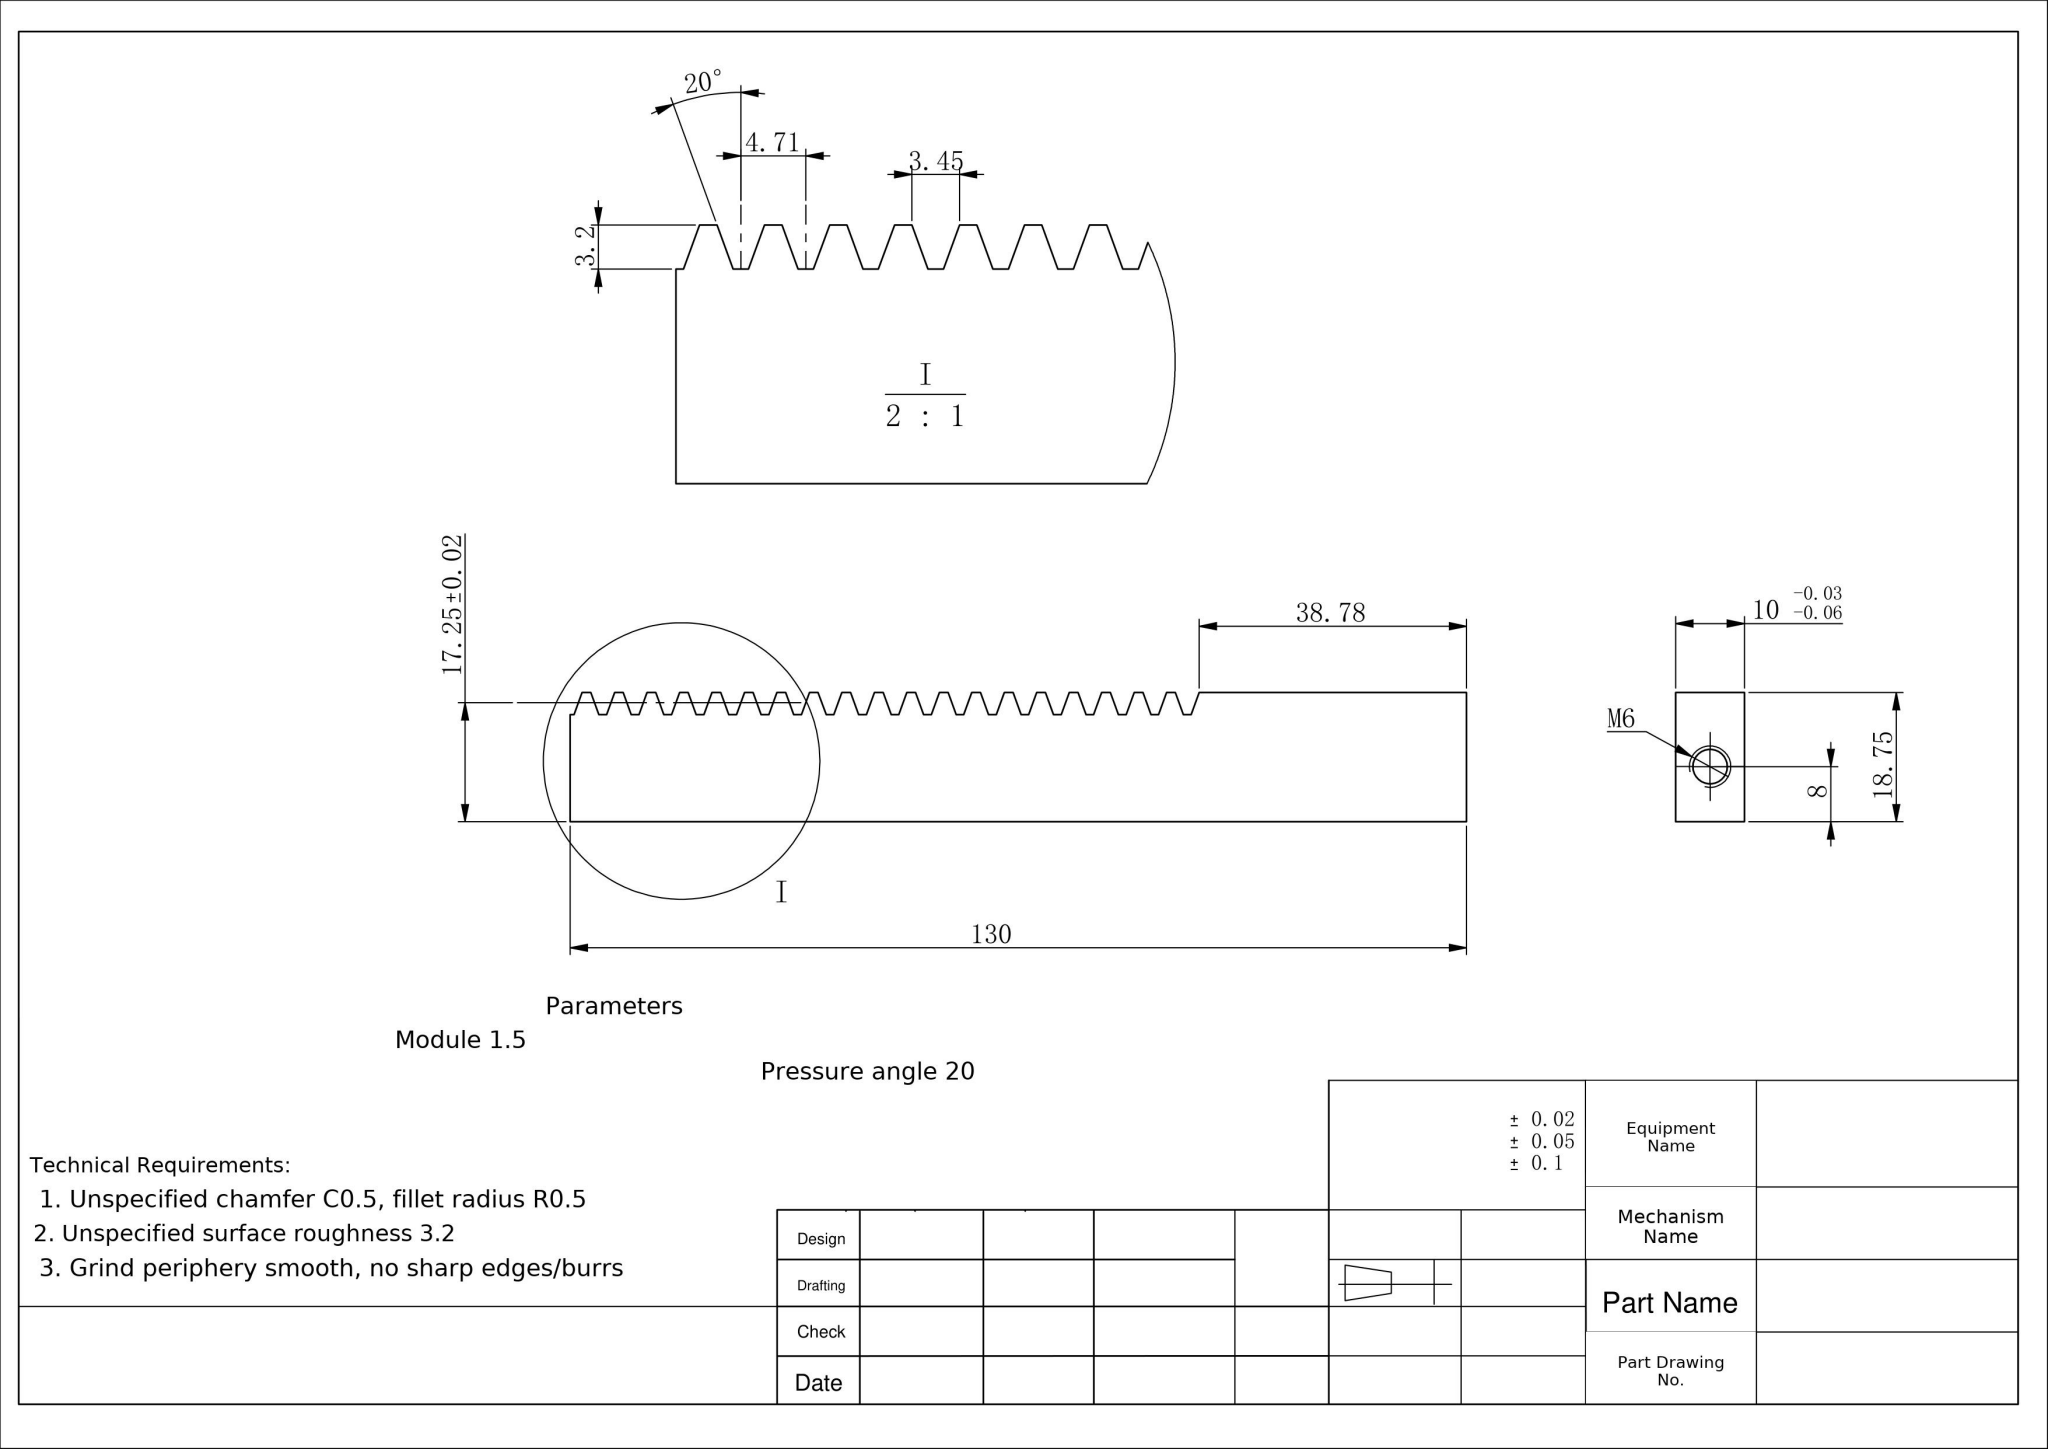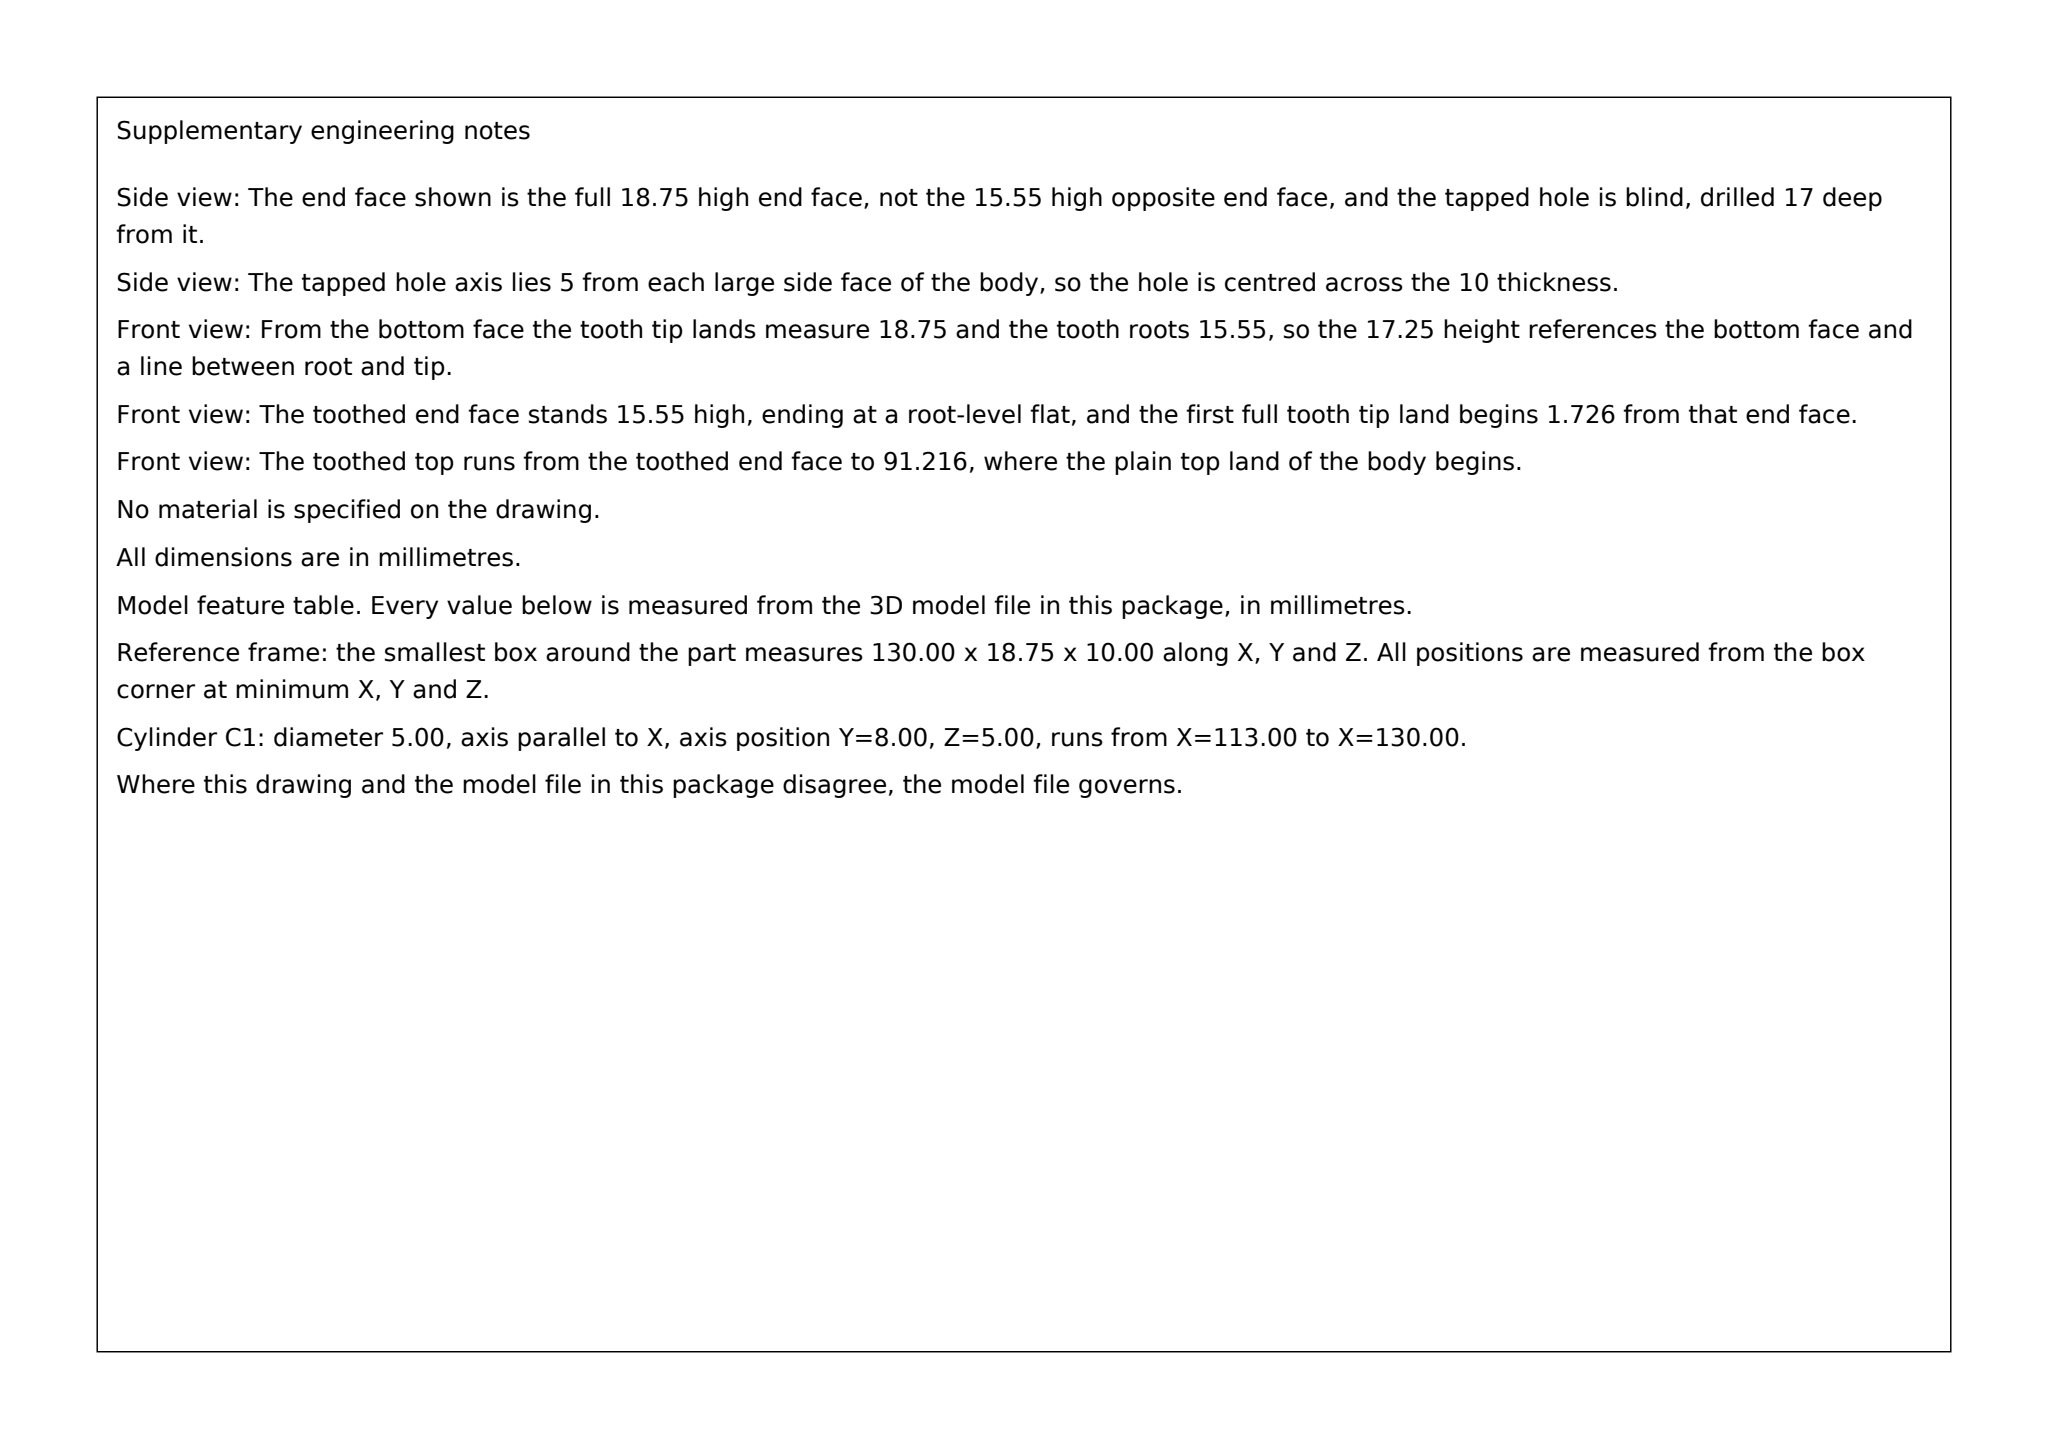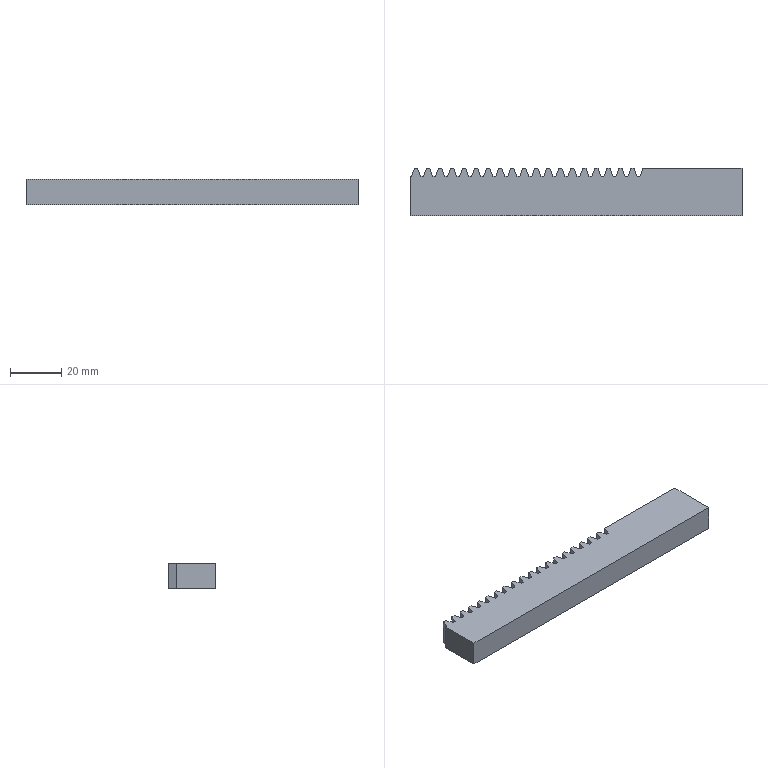Part | SolidWorks | mm | 1 solid | 88 faces | box 130 x 18.75 x 10 mm | volume 22604 mm3 | plane 84 | cylinder 2 | cone 2 | commonest cylinder face diameters 5 x2
Drawing notes:
M6 DP 17 TYP (DRILL PT 118°) | from the solid: cylinders [5.0,'x',[null,8.0,5.0],17.0,2]; cones [118.0,5.0,2]
2X M6 DP 17, ONE IN EA END FACE, 8 UP FROM BTM, ON 5 C/L | from the solid: 2 x-axis holes at y=8.0, z=5.0 (width 10 -> C/L 5), faces x=0 & x=130
20 TEETH @ 4.71 PITCH, TOOTHED LG 91.22 FROM LEFT END FACE | from the solid: 20 planes y=15.55 & 20 planes y=18.75 (3.2 depth); 130-38.78=91.22
build123d program:
from build123d import *

# Parameters (mm, degrees)
SKETCH1_W             = 10
SKETCH1_H             = 18.75
BOSS_EXTRUDE1_DEPTH   = 130
CUT_EXTRUDE1_DEPTH    = 132.725
LPATTERN1_COUNT       = 20
LPATTERN1_PITCH       = 4.71
M6_TAPPED_HOLE1_D     = 5
M6_TAPPED_HOLE1_DEPTH = 17
M6_TAPPED_HOLE1_TIP   = 1.502


with BuildPart() as part:
    # Sketch1 → Boss-Extrude1 (new body)
    with BuildSketch(Plane(origin=(0, 0, 0), x_dir=(0, 0, -1), z_dir=(1, 0, 0))):
        with Locations((5, 9.375)):
            Rectangle(SKETCH1_W, SKETCH1_H)
    extrude(amount=BOSS_EXTRUDE1_DEPTH)

    # Sketch2 → Cut-Extrude1 (cut, through all)
    with BuildSketch(Plane.XY):
        Polygon((-0.5613, 15.55), (0.5613, 15.55), (1.726, 18.75), (-1.726, 18.75), align=None)
    cut_extrude1 = extrude(amount=-CUT_EXTRUDE1_DEPTH, mode=Mode.SUBTRACT)

    # LPattern1: Cut-Extrude1 ×20
    with Locations(*[(i * LPATTERN1_PITCH, 0, 0) for i in range(1, LPATTERN1_COUNT)]):
        add(cut_extrude1, mode=Mode.SUBTRACT)

    # M6 Tapped Hole1
    with Locations(Plane(origin=(130, 0, 0), x_dir=(0, 0, -1), z_dir=(1, 0, 0))):
        with Locations((5, 8)):
            Hole(M6_TAPPED_HOLE1_D / 2, depth=M6_TAPPED_HOLE1_DEPTH)
            with Locations((0, 0, -(M6_TAPPED_HOLE1_DEPTH + M6_TAPPED_HOLE1_TIP / 2))):  # 118° drill point
                Cone(0, M6_TAPPED_HOLE1_D / 2, M6_TAPPED_HOLE1_TIP, mode=Mode.SUBTRACT)


solid = part.part